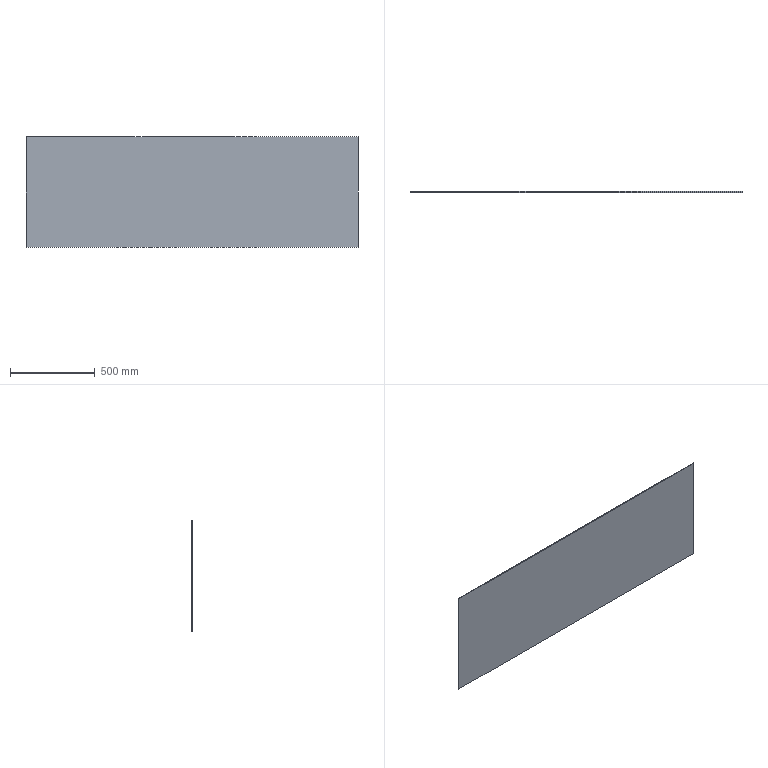Component | SolidWorks | FrontDoorAssembly-1_PG50FrontDoorGlass-1 | 1 solid | 6 faces | box 1956 x 5 x 651 mm | volume 6366780 mm3 | plane 6
build123d program:
from build123d import *

# Parameters (mm, degrees)
SKETCH1_W           = 1956
SKETCH1_H           = 651
BOSS_EXTRUDE1_DEPTH = 5


with BuildPart() as part:
    # Sketch1 → Boss-Extrude1 (new body)
    with BuildSketch(Plane.XY):
        Rectangle(SKETCH1_W, SKETCH1_H)
    extrude(amount=BOSS_EXTRUDE1_DEPTH)


solid = part.part

# Placed as in the assembly
solid = solid.moved(Location((-118.186, -276.799, 0.004001), (90, 0, 0)))
STEP:
#1=CARTESIAN_POINT('',(-43.157,-11.094,-12.815));
#2=VERTEX_POINT('',#1);
#3=CARTESIAN_POINT('',(-43.157,-11.094,12.815));
#4=VERTEX_POINT('',#3);
#5=CARTESIAN_POINT('',(-43.157,-11.094,12.815));
#6=DIRECTION('',(0.,0.,1.));
#7=VECTOR('',#6,39.37);
#8=LINE('',#5,#7);
#9=EDGE_CURVE('',#2,#4,#8,.T.);
#10=ORIENTED_EDGE('',*,*,#9,.T.);
#11=CARTESIAN_POINT('',(-43.157,-10.898,12.815));
#12=VERTEX_POINT('',#11);
#13=CARTESIAN_POINT('',(-43.157,-10.898,12.815));
#14=DIRECTION('',(0.,-1.,-0.));
#15=VECTOR('',#14,39.37);
#16=LINE('',#13,#15);
#17=EDGE_CURVE('',#12,#4,#16,.T.);
#18=ORIENTED_EDGE('',*,*,#17,.F.);
#19=CARTESIAN_POINT('',(-43.157,-10.898,-12.815));
#20=VERTEX_POINT('',#19);
#21=CARTESIAN_POINT('',(-43.157,-10.898,12.815));
#22=DIRECTION('',(0.,0.,1.));
#23=VECTOR('',#22,39.37);
#24=LINE('',#21,#23);
#25=EDGE_CURVE('',#20,#12,#24,.T.);
#26=ORIENTED_EDGE('',*,*,#25,.F.);
#27=CARTESIAN_POINT('',(-43.157,-10.898,-12.815));
#28=DIRECTION('',(0.,-1.,-0.));
#29=VECTOR('',#28,39.37);
#30=LINE('',#27,#29);
#31=EDGE_CURVE('',#20,#2,#30,.T.);
#32=ORIENTED_EDGE('',*,*,#31,.T.);
#33=EDGE_LOOP('',(#10,#18,#26,#32));
#34=FACE_OUTER_BOUND('',#33,.T.);
#35=CARTESIAN_POINT('',(-43.157,-10.898,12.815));
#36=DIRECTION('',(1.,0.,-0.));
#37=DIRECTION('',(0.,-1.,-0.));
#38=AXIS2_PLACEMENT_3D('',#35,#36,#37);
#39=PLANE('',#38);
#40=ADVANCED_FACE('',(#34),#39,.F.);
#41=CARTESIAN_POINT('',(33.851,-11.094,12.815));
#42=VERTEX_POINT('',#41);
#43=CARTESIAN_POINT('',(33.851,-11.094,12.815));
#44=DIRECTION('',(1.,0.,-0.));
#45=VECTOR('',#44,39.37);
#46=LINE('',#43,#45);
#47=EDGE_CURVE('',#4,#42,#46,.T.);
#48=ORIENTED_EDGE('',*,*,#47,.T.);
#49=CARTESIAN_POINT('',(33.851,-10.898,12.815));
#50=VERTEX_POINT('',#49);
#51=CARTESIAN_POINT('',(33.851,-10.898,12.815));
#52=DIRECTION('',(0.,-1.,-0.));
#53=VECTOR('',#52,39.37);
#54=LINE('',#51,#53);
#55=EDGE_CURVE('',#50,#42,#54,.T.);
#56=ORIENTED_EDGE('',*,*,#55,.F.);
#57=CARTESIAN_POINT('',(33.851,-10.898,12.815));
#58=DIRECTION('',(1.,0.,-0.));
#59=VECTOR('',#58,39.37);
#60=LINE('',#57,#59);
#61=EDGE_CURVE('',#12,#50,#60,.T.);
#62=ORIENTED_EDGE('',*,*,#61,.F.);
#63=ORIENTED_EDGE('',*,*,#17,.T.);
#64=EDGE_LOOP('',(#48,#56,#62,#63));
#65=FACE_OUTER_BOUND('',#64,.T.);
#66=CARTESIAN_POINT('',(33.851,-10.898,12.815));
#67=DIRECTION('',(-0.,-0.,-1.));
#68=DIRECTION('',(-1.,-0.,0.));
#69=AXIS2_PLACEMENT_3D('',#66,#67,#68);
#70=PLANE('',#69);
#71=ADVANCED_FACE('',(#65),#70,.F.);
#72=CARTESIAN_POINT('',(33.851,-11.094,-12.815));
#73=VERTEX_POINT('',#72);
#74=CARTESIAN_POINT('',(33.851,-11.094,12.815));
#75=DIRECTION('',(-0.,-0.,-1.));
#76=VECTOR('',#75,39.37);
#77=LINE('',#74,#76);
#78=EDGE_CURVE('',#42,#73,#77,.T.);
#79=ORIENTED_EDGE('',*,*,#78,.T.);
#80=CARTESIAN_POINT('',(33.851,-10.898,-12.815));
#81=VERTEX_POINT('',#80);
#82=CARTESIAN_POINT('',(33.851,-10.898,-12.815));
#83=DIRECTION('',(0.,-1.,-0.));
#84=VECTOR('',#83,39.37);
#85=LINE('',#82,#84);
#86=EDGE_CURVE('',#81,#73,#85,.T.);
#87=ORIENTED_EDGE('',*,*,#86,.F.);
#88=CARTESIAN_POINT('',(33.851,-10.898,12.815));
#89=DIRECTION('',(-0.,-0.,-1.));
#90=VECTOR('',#89,39.37);
#91=LINE('',#88,#90);
#92=EDGE_CURVE('',#50,#81,#91,.T.);
#93=ORIENTED_EDGE('',*,*,#92,.F.);
#94=ORIENTED_EDGE('',*,*,#55,.T.);
#95=EDGE_LOOP('',(#79,#87,#93,#94));
#96=FACE_OUTER_BOUND('',#95,.T.);
#97=CARTESIAN_POINT('',(33.851,-10.898,12.815));
#98=DIRECTION('',(-1.,-0.,0.));
#99=DIRECTION('',(-0.,1.,0.));
#100=AXIS2_PLACEMENT_3D('',#97,#98,#99);
#101=PLANE('',#100);
#102=ADVANCED_FACE('',(#96),#101,.F.);
#103=CARTESIAN_POINT('',(33.851,-11.094,-12.815));
#104=DIRECTION('',(-1.,-0.,0.));
#105=VECTOR('',#104,39.37);
#106=LINE('',#103,#105);
#107=EDGE_CURVE('',#73,#2,#106,.T.);
#108=ORIENTED_EDGE('',*,*,#107,.T.);
#109=ORIENTED_EDGE('',*,*,#31,.F.);
#110=CARTESIAN_POINT('',(33.851,-10.898,-12.815));
#111=DIRECTION('',(-1.,-0.,0.));
#112=VECTOR('',#111,39.37);
#113=LINE('',#110,#112);
#114=EDGE_CURVE('',#81,#20,#113,.T.);
#115=ORIENTED_EDGE('',*,*,#114,.F.);
#116=ORIENTED_EDGE('',*,*,#86,.T.);
#117=EDGE_LOOP('',(#108,#109,#115,#116));
#118=FACE_OUTER_BOUND('',#117,.T.);
#119=CARTESIAN_POINT('',(33.851,-10.898,-12.815));
#120=DIRECTION('',(0.,0.,1.));
#121=DIRECTION('',(1.,0.,-0.));
#122=AXIS2_PLACEMENT_3D('',#119,#120,#121);
#123=PLANE('',#122);
#124=ADVANCED_FACE('',(#118),#123,.F.);
#125=ORIENTED_EDGE('',*,*,#25,.T.);
#126=ORIENTED_EDGE('',*,*,#61,.T.);
#127=ORIENTED_EDGE('',*,*,#92,.T.);
#128=ORIENTED_EDGE('',*,*,#114,.T.);
#129=EDGE_LOOP('',(#125,#126,#127,#128));
#130=FACE_OUTER_BOUND('',#129,.T.);
#131=CARTESIAN_POINT('',(-4.653,-10.898,0.0001575));
#132=DIRECTION('',(-0.,1.,0.));
#133=DIRECTION('',(1.,0.,-0.));
#134=AXIS2_PLACEMENT_3D('',#131,#132,#133);
#135=PLANE('',#134);
#136=ADVANCED_FACE('',(#130),#135,.T.);
#137=ORIENTED_EDGE('',*,*,#9,.F.);
#138=ORIENTED_EDGE('',*,*,#107,.F.);
#139=ORIENTED_EDGE('',*,*,#78,.F.);
#140=ORIENTED_EDGE('',*,*,#47,.F.);
#141=EDGE_LOOP('',(#137,#138,#139,#140));
#142=FACE_OUTER_BOUND('',#141,.T.);
#143=CARTESIAN_POINT('',(-4.653,-11.094,0.0001575));
#144=DIRECTION('',(-0.,1.,0.));
#145=DIRECTION('',(1.,0.,-0.));
#146=AXIS2_PLACEMENT_3D('',#143,#144,#145);
#147=PLANE('',#146);
#148=ADVANCED_FACE('',(#142),#147,.F.);
#149=CLOSED_SHELL('',(#40,#71,#102,#124,#136,#148));
#150=MANIFOLD_SOLID_BREP('',#149);
#151=CARTESIAN_POINT('',(0.,0.,0.));
#152=DIRECTION('',(0.,0.,1.));
#153=DIRECTION('',(1.,0.,0.));
#154=AXIS2_PLACEMENT_3D('',#151,#152,#153);
#155=(LENGTH_UNIT()NAMED_UNIT(*)SI_UNIT($,.METRE.));
#156=LENGTH_MEASURE_WITH_UNIT(LENGTH_MEASURE(0.0254),#155);
#157=DIMENSIONAL_EXPONENTS(1.,0.,0.,0.,0.,0.,0.);
#158=(CONVERSION_BASED_UNIT('',#156)LENGTH_UNIT()NAMED_UNIT(#157));
#159=UNCERTAINTY_MEASURE_WITH_UNIT(LENGTH_MEASURE(0.00001),#158,'','');
#160=(NAMED_UNIT(*)PLANE_ANGLE_UNIT()SI_UNIT($,.RADIAN.));
#161=(NAMED_UNIT(*)SI_UNIT($,.STERADIAN.)SOLID_ANGLE_UNIT());
#162=(GEOMETRIC_REPRESENTATION_CONTEXT(3)GLOBAL_UNCERTAINTY_ASSIGNED_CONTEXT((#159))GLOBAL_UNIT_ASSIGNED_CONTEXT((#158,#160,#161))REPRESENTATION_CONTEXT('',''));
#163=ADVANCED_BREP_SHAPE_REPRESENTATION('',(#150,#154),#162);
#164=COLOUR_RGB('',0.7922,0.8196,0.9333);
#165=FILL_AREA_STYLE_COLOUR('',#164);
#166=FILL_AREA_STYLE('',(#165));
#167=SURFACE_STYLE_FILL_AREA(#166);
#168=SURFACE_SIDE_STYLE('',(#167));
#169=SURFACE_STYLE_USAGE(.BOTH.,#168);
#170=PRESENTATION_STYLE_ASSIGNMENT((#169));
#171=STYLED_ITEM('',(#170),#150);
#172=PRESENTATION_LAYER_ASSIGNMENT('','',(#171));
#173=(LENGTH_UNIT()NAMED_UNIT(*)SI_UNIT($,.METRE.));
#174=LENGTH_MEASURE_WITH_UNIT(LENGTH_MEASURE(0.0254),#173);
#175=DIMENSIONAL_EXPONENTS(1.,0.,0.,0.,0.,0.,0.);
#176=(CONVERSION_BASED_UNIT('',#174)LENGTH_UNIT()NAMED_UNIT(#175));
#177=UNCERTAINTY_MEASURE_WITH_UNIT(LENGTH_MEASURE(0.00001),#176,'','');
#178=(NAMED_UNIT(*)PLANE_ANGLE_UNIT()SI_UNIT($,.RADIAN.));
#179=(NAMED_UNIT(*)SI_UNIT($,.STERADIAN.)SOLID_ANGLE_UNIT());
#180=(GEOMETRIC_REPRESENTATION_CONTEXT(3)GLOBAL_UNCERTAINTY_ASSIGNED_CONTEXT((#177))GLOBAL_UNIT_ASSIGNED_CONTEXT((#176,#178,#179))REPRESENTATION_CONTEXT('',''));
#181=MECHANICAL_DESIGN_GEOMETRIC_PRESENTATION_REPRESENTATION('',(#171),#180);